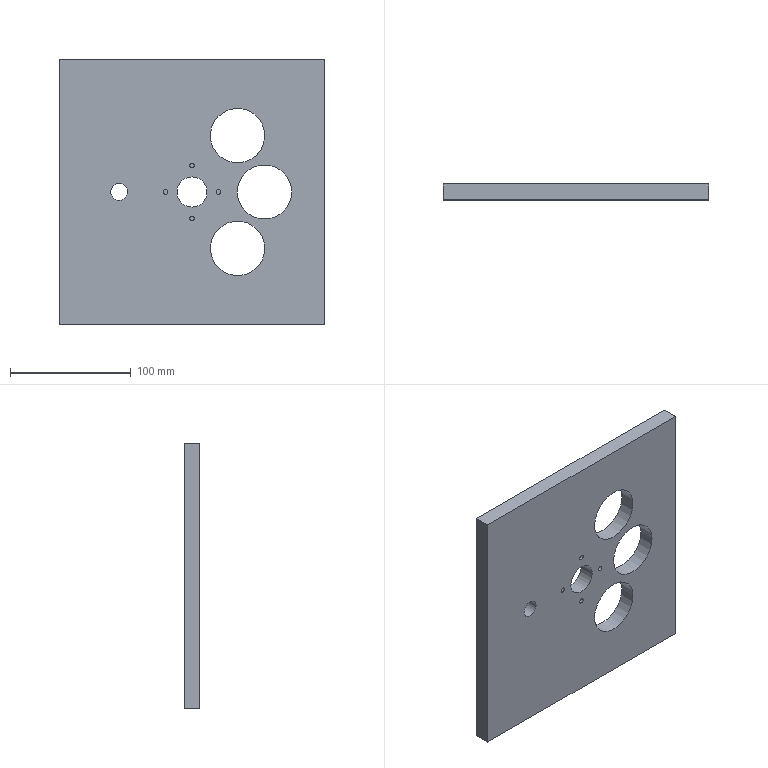Component | NX | VALVE_BODY | 1 solid | 23 faces | volume 557484 mm3 | plane 12 | cylinder 11 | commonest cylinder face diameters 4 x4 45 x3 8 x2 14 x1 25 x1